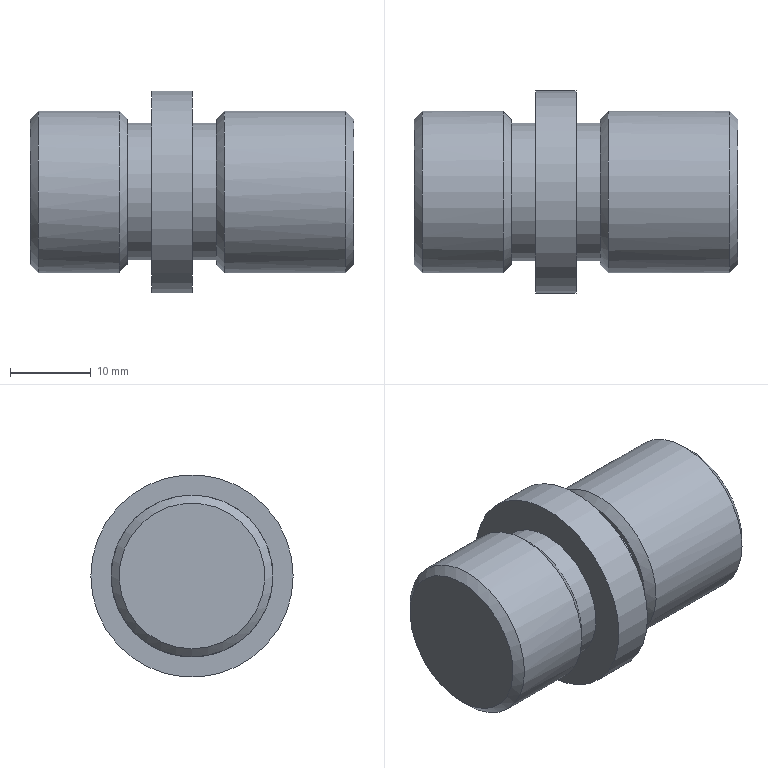Component | NX | MANDREL | 1 solid | 15 faces | box 40 x 25 x 25 mm | volume 12805 mm3 | plane 6 | cylinder 5 | cone 4 | commonest cylinder face diameters 17 x2 20 x2 25 x1
STEP:
#1=CARTESIAN_POINT('',(0.,0.,0.));
#2=DIRECTION('',(0.,0.,1.));
#3=DIRECTION('',(1.,0.,0.));
#4=AXIS2_PLACEMENT_3D('',#1,#2,#3);
#5=CARTESIAN_POINT('',(-22.,12.5,-57.));
#6=VERTEX_POINT('',#5);
#7=CARTESIAN_POINT('',(-22.,0.,-57.));
#8=DIRECTION('',(1.,0.,0.));
#9=DIRECTION('',(0.,1.,0.));
#10=AXIS2_PLACEMENT_3D('',#7,#8,#9);
#11=CIRCLE('',#10,12.5);
#12=CARTESIAN_POINT('',(-22.,0.,-57.));
#13=DIRECTION('',(-1.,0.,0.));
#14=DIRECTION('',(0.,0.,1.));
#15=AXIS2_PLACEMENT_3D('',#12,#13,#14);
#16=CYLINDRICAL_SURFACE('',#15,12.5);
#17=CARTESIAN_POINT('',(7.854,0.));
#18=DIRECTION('',(-1.,0.));
#19=VECTOR('',#18,1.);
#20=LINE('',#17,#19);
#21=(GEOMETRIC_REPRESENTATION_CONTEXT(2)PARAMETRIC_REPRESENTATION_CONTEXT()REPRESENTATION_CONTEXT('',''));
#22=DEFINITIONAL_REPRESENTATION('',(#20),#21);
#23=PCURVE('',#16,#22);
#24=CARTESIAN_POINT('',(-22.,0.,-57.));
#25=DIRECTION('',(1.,0.,0.));
#26=DIRECTION('',(0.,0.,-1.));
#27=AXIS2_PLACEMENT_3D('',#24,#25,#26);
#28=PLANE('',#27);
#29=CARTESIAN_POINT('',(0.,0.));
#30=DIRECTION('',(0.,1.));
#31=AXIS2_PLACEMENT_2D('',#29,#30);
#32=CIRCLE('',#31,12.5);
#33=(GEOMETRIC_REPRESENTATION_CONTEXT(2)PARAMETRIC_REPRESENTATION_CONTEXT()REPRESENTATION_CONTEXT('',''));
#34=DEFINITIONAL_REPRESENTATION('',(#32),#33);
#35=PCURVE('',#28,#34);
#36=SURFACE_CURVE('',#11,(#23,#35),.PCURVE_S1.);
#37=EDGE_CURVE('',#6,#6,#36,.T.);
#38=ORIENTED_EDGE('',*,*,#37,.F.);
#39=CARTESIAN_POINT('',(-27.,12.5,-57.));
#40=VERTEX_POINT('',#39);
#41=CARTESIAN_POINT('',(-22.,12.5,-57.));
#42=CARTESIAN_POINT('',(-27.,12.5,-57.));
#43=B_SPLINE_CURVE_WITH_KNOTS('',1,(#41,#42),.UNSPECIFIED.,.F.,.F.,(2,2),(0.,5.),.PIECEWISE_BEZIER_KNOTS.);
#44=CARTESIAN_POINT('',(7.854,0.));
#45=DIRECTION('',(0.,1.));
#46=VECTOR('',#45,1.);
#47=LINE('',#44,#46);
#48=(GEOMETRIC_REPRESENTATION_CONTEXT(2)PARAMETRIC_REPRESENTATION_CONTEXT()REPRESENTATION_CONTEXT('',''));
#49=DEFINITIONAL_REPRESENTATION('',(#47),#48);
#50=PCURVE('',#16,#49);
#51=CARTESIAN_POINT('',(1.571,0.));
#52=DIRECTION('',(0.,1.));
#53=VECTOR('',#52,1.);
#54=LINE('',#51,#53);
#55=(GEOMETRIC_REPRESENTATION_CONTEXT(2)PARAMETRIC_REPRESENTATION_CONTEXT()REPRESENTATION_CONTEXT('',''));
#56=DEFINITIONAL_REPRESENTATION('',(#54),#55);
#57=PCURVE('',#16,#56);
#58=SEAM_CURVE('',#43,(#50,#57),.PCURVE_S1.);
#59=EDGE_CURVE('',#6,#40,#58,.T.);
#60=ORIENTED_EDGE('',*,*,#59,.T.);
#61=CARTESIAN_POINT('',(-27.,0.,-57.));
#62=DIRECTION('',(1.,0.,0.));
#63=DIRECTION('',(0.,1.,0.));
#64=AXIS2_PLACEMENT_3D('',#61,#62,#63);
#65=CIRCLE('',#64,12.5);
#66=CARTESIAN_POINT('',(7.854,5.));
#67=DIRECTION('',(-1.,0.));
#68=VECTOR('',#67,1.);
#69=LINE('',#66,#68);
#70=(GEOMETRIC_REPRESENTATION_CONTEXT(2)PARAMETRIC_REPRESENTATION_CONTEXT()REPRESENTATION_CONTEXT('',''));
#71=DEFINITIONAL_REPRESENTATION('',(#69),#70);
#72=PCURVE('',#16,#71);
#73=CARTESIAN_POINT('',(-27.,0.,-57.));
#74=DIRECTION('',(1.,0.,0.));
#75=DIRECTION('',(0.,0.,-1.));
#76=AXIS2_PLACEMENT_3D('',#73,#74,#75);
#77=PLANE('',#76);
#78=CARTESIAN_POINT('',(0.,0.));
#79=DIRECTION('',(0.,1.));
#80=AXIS2_PLACEMENT_2D('',#78,#79);
#81=CIRCLE('',#80,12.5);
#82=(GEOMETRIC_REPRESENTATION_CONTEXT(2)PARAMETRIC_REPRESENTATION_CONTEXT()REPRESENTATION_CONTEXT('',''));
#83=DEFINITIONAL_REPRESENTATION('',(#81),#82);
#84=PCURVE('',#77,#83);
#85=SURFACE_CURVE('',#65,(#72,#84),.PCURVE_S1.);
#86=EDGE_CURVE('',#40,#40,#85,.T.);
#87=ORIENTED_EDGE('',*,*,#86,.T.);
#88=ORIENTED_EDGE('',*,*,#59,.F.);
#89=EDGE_LOOP('',(#38,#60,#87,#88));
#90=FACE_BOUND('',#89,.T.);
#91=ADVANCED_FACE('',(#90),#16,.T.);
#92=ORIENTED_EDGE('',*,*,#37,.T.);
#93=EDGE_LOOP('',(#92));
#94=FACE_BOUND('',#93,.T.);
#95=CARTESIAN_POINT('',(-22.,0.,-48.5));
#96=VERTEX_POINT('',#95);
#97=CARTESIAN_POINT('',(-22.,0.,-57.));
#98=DIRECTION('',(-1.,0.,0.));
#99=DIRECTION('',(0.,0.,1.));
#100=AXIS2_PLACEMENT_3D('',#97,#98,#99);
#101=CIRCLE('',#100,8.5);
#102=CARTESIAN_POINT('',(-8.5,0.));
#103=CARTESIAN_POINT('',(-8.5,14.722));
#104=CARTESIAN_POINT('',(4.25,7.361));
#105=CARTESIAN_POINT('',(17.,0.));
#106=CARTESIAN_POINT('',(4.25,-7.361));
#107=CARTESIAN_POINT('',(-8.5,-14.722));
#108=CARTESIAN_POINT('',(-8.5,0.));
#109=(BOUNDED_CURVE()B_SPLINE_CURVE(2,(#102,#103,#104,#105,#106,#107,#108),.UNSPECIFIED.,.T.,.F.)B_SPLINE_CURVE_WITH_KNOTS((1,2,2,2,2,1),(-2.094,0.,2.094,4.189,6.283,8.378),.UNSPECIFIED.)CURVE()GEOMETRIC_REPRESENTATION_ITEM()RATIONAL_B_SPLINE_CURVE((1.,0.5,1.,0.5,1.,0.5,1.))REPRESENTATION_ITEM(''));
#110=(GEOMETRIC_REPRESENTATION_CONTEXT(2)PARAMETRIC_REPRESENTATION_CONTEXT()REPRESENTATION_CONTEXT('',''));
#111=DEFINITIONAL_REPRESENTATION('',(#109),#110);
#112=PCURVE('',#28,#111);
#113=CARTESIAN_POINT('',(-20.5,0.,-57.));
#114=DIRECTION('',(-1.,0.,0.));
#115=DIRECTION('',(0.,0.,1.));
#116=AXIS2_PLACEMENT_3D('',#113,#114,#115);
#117=CYLINDRICAL_SURFACE('',#116,8.5);
#118=CARTESIAN_POINT('',(0.,1.5));
#119=DIRECTION('',(1.,0.));
#120=VECTOR('',#119,1.);
#121=LINE('',#118,#120);
#122=(GEOMETRIC_REPRESENTATION_CONTEXT(2)PARAMETRIC_REPRESENTATION_CONTEXT()REPRESENTATION_CONTEXT('',''));
#123=DEFINITIONAL_REPRESENTATION('',(#121),#122);
#124=PCURVE('',#117,#123);
#125=SURFACE_CURVE('',#101,(#112,#124),.PCURVE_S1.);
#126=EDGE_CURVE('',#96,#96,#125,.T.);
#127=ORIENTED_EDGE('',*,*,#126,.T.);
#128=EDGE_LOOP('',(#127));
#129=FACE_BOUND('',#128,.T.);
#130=ADVANCED_FACE('',(#94,#129),#28,.T.);
#131=ORIENTED_EDGE('',*,*,#86,.F.);
#132=EDGE_LOOP('',(#131));
#133=FACE_BOUND('',#132,.T.);
#134=CARTESIAN_POINT('',(-27.,0.,-48.5));
#135=VERTEX_POINT('',#134);
#136=CARTESIAN_POINT('',(-27.,0.,-57.));
#137=DIRECTION('',(-1.,0.,0.));
#138=DIRECTION('',(0.,0.,1.));
#139=AXIS2_PLACEMENT_3D('',#136,#137,#138);
#140=CIRCLE('',#139,8.5);
#141=CARTESIAN_POINT('',(-8.5,0.));
#142=CARTESIAN_POINT('',(-8.5,14.722));
#143=CARTESIAN_POINT('',(4.25,7.361));
#144=CARTESIAN_POINT('',(17.,0.));
#145=CARTESIAN_POINT('',(4.25,-7.361));
#146=CARTESIAN_POINT('',(-8.5,-14.722));
#147=CARTESIAN_POINT('',(-8.5,0.));
#148=(BOUNDED_CURVE()B_SPLINE_CURVE(2,(#141,#142,#143,#144,#145,#146,#147),.UNSPECIFIED.,.T.,.F.)B_SPLINE_CURVE_WITH_KNOTS((1,2,2,2,2,1),(-2.094,0.,2.094,4.189,6.283,8.378),.UNSPECIFIED.)CURVE()GEOMETRIC_REPRESENTATION_ITEM()RATIONAL_B_SPLINE_CURVE((1.,0.5,1.,0.5,1.,0.5,1.))REPRESENTATION_ITEM(''));
#149=(GEOMETRIC_REPRESENTATION_CONTEXT(2)PARAMETRIC_REPRESENTATION_CONTEXT()REPRESENTATION_CONTEXT('',''));
#150=DEFINITIONAL_REPRESENTATION('',(#148),#149);
#151=PCURVE('',#77,#150);
#152=CARTESIAN_POINT('',(-28.5,0.,-57.));
#153=DIRECTION('',(-1.,0.,0.));
#154=DIRECTION('',(0.,0.,1.));
#155=AXIS2_PLACEMENT_3D('',#152,#153,#154);
#156=CYLINDRICAL_SURFACE('',#155,8.5);
#157=CARTESIAN_POINT('',(0.,-1.5));
#158=DIRECTION('',(1.,0.));
#159=VECTOR('',#158,1.);
#160=LINE('',#157,#159);
#161=(GEOMETRIC_REPRESENTATION_CONTEXT(2)PARAMETRIC_REPRESENTATION_CONTEXT()REPRESENTATION_CONTEXT('',''));
#162=DEFINITIONAL_REPRESENTATION('',(#160),#161);
#163=PCURVE('',#156,#162);
#164=SURFACE_CURVE('',#140,(#151,#163),.PCURVE_S1.);
#165=EDGE_CURVE('',#135,#135,#164,.T.);
#166=ORIENTED_EDGE('',*,*,#165,.F.);
#167=EDGE_LOOP('',(#166));
#168=FACE_BOUND('',#167,.T.);
#169=ADVANCED_FACE('',(#133,#168),#77,.F.);
#170=CARTESIAN_POINT('',(-30.,0.,-48.));
#171=VERTEX_POINT('',#170);
#172=CARTESIAN_POINT('',(-30.,0.,-57.));
#173=DIRECTION('',(1.,0.,0.));
#174=DIRECTION('',(0.,0.,1.));
#175=AXIS2_PLACEMENT_3D('',#172,#173,#174);
#176=CIRCLE('',#175,9.);
#177=CARTESIAN_POINT('',(-30.,0.,-57.));
#178=DIRECTION('',(-1.,0.,0.));
#179=DIRECTION('',(0.,0.,1.));
#180=AXIS2_PLACEMENT_3D('',#177,#178,#179);
#181=PLANE('',#180);
#182=CARTESIAN_POINT('',(9.,0.));
#183=CARTESIAN_POINT('',(9.,-15.588));
#184=CARTESIAN_POINT('',(-4.5,-7.794));
#185=CARTESIAN_POINT('',(-18.,-0.));
#186=CARTESIAN_POINT('',(-4.5,7.794));
#187=CARTESIAN_POINT('',(9.,15.588));
#188=CARTESIAN_POINT('',(9.,0.));
#189=(BOUNDED_CURVE()B_SPLINE_CURVE(2,(#182,#183,#184,#185,#186,#187,#188),.UNSPECIFIED.,.T.,.F.)B_SPLINE_CURVE_WITH_KNOTS((1,2,2,2,2,1),(-2.094,0.,2.094,4.189,6.283,8.378),.UNSPECIFIED.)CURVE()GEOMETRIC_REPRESENTATION_ITEM()RATIONAL_B_SPLINE_CURVE((1.,0.5,1.,0.5,1.,0.5,1.))REPRESENTATION_ITEM(''));
#190=(GEOMETRIC_REPRESENTATION_CONTEXT(2)PARAMETRIC_REPRESENTATION_CONTEXT()REPRESENTATION_CONTEXT('',''));
#191=DEFINITIONAL_REPRESENTATION('',(#189),#190);
#192=PCURVE('',#181,#191);
#193=CARTESIAN_POINT('',(-31.,0.,-57.));
#194=DIRECTION('',(-1.,0.,0.));
#195=DIRECTION('',(0.,0.,1.));
#196=AXIS2_PLACEMENT_3D('',#193,#194,#195);
#197=CONICAL_SURFACE('',#196,10.,0.7854);
#198=CARTESIAN_POINT('',(6.283,-1.));
#199=DIRECTION('',(-1.,0.));
#200=VECTOR('',#199,1.);
#201=LINE('',#198,#200);
#202=(GEOMETRIC_REPRESENTATION_CONTEXT(2)PARAMETRIC_REPRESENTATION_CONTEXT()REPRESENTATION_CONTEXT('',''));
#203=DEFINITIONAL_REPRESENTATION('',(#201),#202);
#204=PCURVE('',#197,#203);
#205=SURFACE_CURVE('',#176,(#192,#204),.PCURVE_S1.);
#206=EDGE_CURVE('',#171,#171,#205,.T.);
#207=ORIENTED_EDGE('',*,*,#206,.T.);
#208=EDGE_LOOP('',(#207));
#209=FACE_BOUND('',#208,.T.);
#210=CARTESIAN_POINT('',(-30.,0.,-48.5));
#211=VERTEX_POINT('',#210);
#212=CARTESIAN_POINT('',(-30.,0.,-57.));
#213=DIRECTION('',(1.,0.,0.));
#214=DIRECTION('',(0.,0.,1.));
#215=AXIS2_PLACEMENT_3D('',#212,#213,#214);
#216=CIRCLE('',#215,8.5);
#217=CARTESIAN_POINT('',(8.5,0.));
#218=CARTESIAN_POINT('',(8.5,-14.722));
#219=CARTESIAN_POINT('',(-4.25,-7.361));
#220=CARTESIAN_POINT('',(-17.,-0.));
#221=CARTESIAN_POINT('',(-4.25,7.361));
#222=CARTESIAN_POINT('',(8.5,14.722));
#223=CARTESIAN_POINT('',(8.5,0.));
#224=(BOUNDED_CURVE()B_SPLINE_CURVE(2,(#217,#218,#219,#220,#221,#222,#223),.UNSPECIFIED.,.T.,.F.)B_SPLINE_CURVE_WITH_KNOTS((1,2,2,2,2,1),(-2.094,0.,2.094,4.189,6.283,8.378),.UNSPECIFIED.)CURVE()GEOMETRIC_REPRESENTATION_ITEM()RATIONAL_B_SPLINE_CURVE((1.,0.5,1.,0.5,1.,0.5,1.))REPRESENTATION_ITEM(''));
#225=(GEOMETRIC_REPRESENTATION_CONTEXT(2)PARAMETRIC_REPRESENTATION_CONTEXT()REPRESENTATION_CONTEXT('',''));
#226=DEFINITIONAL_REPRESENTATION('',(#224),#225);
#227=PCURVE('',#181,#226);
#228=CARTESIAN_POINT('',(6.283,1.5));
#229=DIRECTION('',(-1.,0.));
#230=VECTOR('',#229,1.);
#231=LINE('',#228,#230);
#232=(GEOMETRIC_REPRESENTATION_CONTEXT(2)PARAMETRIC_REPRESENTATION_CONTEXT()REPRESENTATION_CONTEXT('',''));
#233=DEFINITIONAL_REPRESENTATION('',(#231),#232);
#234=PCURVE('',#156,#233);
#235=SURFACE_CURVE('',#216,(#227,#234),.PCURVE_S1.);
#236=EDGE_CURVE('',#211,#211,#235,.T.);
#237=ORIENTED_EDGE('',*,*,#236,.F.);
#238=EDGE_LOOP('',(#237));
#239=FACE_BOUND('',#238,.T.);
#240=ADVANCED_FACE('',(#209,#239),#181,.F.);
#241=ORIENTED_EDGE('',*,*,#236,.T.);
#242=CARTESIAN_POINT('',(-27.,-0.,-48.5));
#243=CARTESIAN_POINT('',(-30.,-0.,-48.5));
#244=B_SPLINE_CURVE_WITH_KNOTS('',1,(#242,#243),.UNSPECIFIED.,.F.,.F.,(2,2),(-1.5,1.5),.PIECEWISE_BEZIER_KNOTS.);
#245=CARTESIAN_POINT('',(0.,0.));
#246=DIRECTION('',(0.,1.));
#247=VECTOR('',#246,1.);
#248=LINE('',#245,#247);
#249=(GEOMETRIC_REPRESENTATION_CONTEXT(2)PARAMETRIC_REPRESENTATION_CONTEXT()REPRESENTATION_CONTEXT('',''));
#250=DEFINITIONAL_REPRESENTATION('',(#248),#249);
#251=PCURVE('',#156,#250);
#252=CARTESIAN_POINT('',(6.283,0.));
#253=DIRECTION('',(0.,1.));
#254=VECTOR('',#253,1.);
#255=LINE('',#252,#254);
#256=(GEOMETRIC_REPRESENTATION_CONTEXT(2)PARAMETRIC_REPRESENTATION_CONTEXT()REPRESENTATION_CONTEXT('',''));
#257=DEFINITIONAL_REPRESENTATION('',(#255),#256);
#258=PCURVE('',#156,#257);
#259=SEAM_CURVE('',#244,(#251,#258),.PCURVE_S1.);
#260=EDGE_CURVE('',#135,#211,#259,.T.);
#261=ORIENTED_EDGE('',*,*,#260,.F.);
#262=ORIENTED_EDGE('',*,*,#165,.T.);
#263=ORIENTED_EDGE('',*,*,#260,.T.);
#264=EDGE_LOOP('',(#241,#261,#262,#263));
#265=FACE_BOUND('',#264,.T.);
#266=ADVANCED_FACE('',(#265),#156,.T.);
#267=CARTESIAN_POINT('',(-42.,0.,-66.));
#268=VERTEX_POINT('',#267);
#269=CARTESIAN_POINT('',(-42.,0.,-57.));
#270=DIRECTION('',(-1.,0.,0.));
#271=DIRECTION('',(0.,0.,-1.));
#272=AXIS2_PLACEMENT_3D('',#269,#270,#271);
#273=CIRCLE('',#272,9.);
#274=CARTESIAN_POINT('',(-42.,0.,-57.));
#275=DIRECTION('',(1.,0.,0.));
#276=DIRECTION('',(0.,0.,-1.));
#277=AXIS2_PLACEMENT_3D('',#274,#275,#276);
#278=PLANE('',#277);
#279=CARTESIAN_POINT('',(9.,0.));
#280=CARTESIAN_POINT('',(9.,-15.588));
#281=CARTESIAN_POINT('',(-4.5,-7.794));
#282=CARTESIAN_POINT('',(-18.,-0.));
#283=CARTESIAN_POINT('',(-4.5,7.794));
#284=CARTESIAN_POINT('',(9.,15.588));
#285=CARTESIAN_POINT('',(9.,0.));
#286=(BOUNDED_CURVE()B_SPLINE_CURVE(2,(#279,#280,#281,#282,#283,#284,#285),.UNSPECIFIED.,.T.,.F.)B_SPLINE_CURVE_WITH_KNOTS((1,2,2,2,2,1),(-2.094,0.,2.094,4.189,6.283,8.378),.UNSPECIFIED.)CURVE()GEOMETRIC_REPRESENTATION_ITEM()RATIONAL_B_SPLINE_CURVE((1.,0.5,1.,0.5,1.,0.5,1.))REPRESENTATION_ITEM(''));
#287=(GEOMETRIC_REPRESENTATION_CONTEXT(2)PARAMETRIC_REPRESENTATION_CONTEXT()REPRESENTATION_CONTEXT('',''));
#288=DEFINITIONAL_REPRESENTATION('',(#286),#287);
#289=PCURVE('',#278,#288);
#290=CARTESIAN_POINT('',(-41.,0.,-57.));
#291=DIRECTION('',(1.,0.,0.));
#292=DIRECTION('',(0.,0.,-1.));
#293=AXIS2_PLACEMENT_3D('',#290,#291,#292);
#294=CONICAL_SURFACE('',#293,10.,0.7854);
#295=CARTESIAN_POINT('',(6.283,-1.));
#296=DIRECTION('',(-1.,0.));
#297=VECTOR('',#296,1.);
#298=LINE('',#295,#297);
#299=(GEOMETRIC_REPRESENTATION_CONTEXT(2)PARAMETRIC_REPRESENTATION_CONTEXT()REPRESENTATION_CONTEXT('',''));
#300=DEFINITIONAL_REPRESENTATION('',(#298),#299);
#301=PCURVE('',#294,#300);
#302=SURFACE_CURVE('',#273,(#289,#301),.PCURVE_S1.);
#303=EDGE_CURVE('',#268,#268,#302,.T.);
#304=ORIENTED_EDGE('',*,*,#303,.T.);
#305=EDGE_LOOP('',(#304));
#306=FACE_BOUND('',#305,.T.);
#307=ADVANCED_FACE('',(#306),#278,.F.);
#308=CARTESIAN_POINT('',(-31.,0.,-47.));
#309=VERTEX_POINT('',#308);
#310=CARTESIAN_POINT('',(-31.,0.,-57.));
#311=DIRECTION('',(-1.,0.,0.));
#312=DIRECTION('',(0.,0.,1.));
#313=AXIS2_PLACEMENT_3D('',#310,#311,#312);
#314=CIRCLE('',#313,10.);
#315=CARTESIAN_POINT('',(-27.,0.,-57.));
#316=DIRECTION('',(-1.,0.,0.));
#317=DIRECTION('',(0.,0.,1.));
#318=AXIS2_PLACEMENT_3D('',#315,#316,#317);
#319=CYLINDRICAL_SURFACE('',#318,10.);
#320=CARTESIAN_POINT('',(0.,4.));
#321=DIRECTION('',(1.,0.));
#322=VECTOR('',#321,1.);
#323=LINE('',#320,#322);
#324=(GEOMETRIC_REPRESENTATION_CONTEXT(2)PARAMETRIC_REPRESENTATION_CONTEXT()REPRESENTATION_CONTEXT('',''));
#325=DEFINITIONAL_REPRESENTATION('',(#323),#324);
#326=PCURVE('',#319,#325);
#327=CARTESIAN_POINT('',(0.,0.));
#328=DIRECTION('',(1.,0.));
#329=VECTOR('',#328,1.);
#330=LINE('',#327,#329);
#331=(GEOMETRIC_REPRESENTATION_CONTEXT(2)PARAMETRIC_REPRESENTATION_CONTEXT()REPRESENTATION_CONTEXT('',''));
#332=DEFINITIONAL_REPRESENTATION('',(#330),#331);
#333=PCURVE('',#197,#332);
#334=SURFACE_CURVE('',#314,(#326,#333),.PCURVE_S1.);
#335=EDGE_CURVE('',#309,#309,#334,.T.);
#336=ORIENTED_EDGE('',*,*,#335,.T.);
#337=CARTESIAN_POINT('',(-41.,0.,-47.));
#338=VERTEX_POINT('',#337);
#339=CARTESIAN_POINT('',(-31.,0.,-47.));
#340=CARTESIAN_POINT('',(-41.,0.,-47.));
#341=B_SPLINE_CURVE_WITH_KNOTS('',1,(#339,#340),.UNSPECIFIED.,.F.,.F.,(2,2),(4.,14.),.PIECEWISE_BEZIER_KNOTS.);
#342=CARTESIAN_POINT('',(6.283,0.));
#343=DIRECTION('',(0.,1.));
#344=VECTOR('',#343,1.);
#345=LINE('',#342,#344);
#346=(GEOMETRIC_REPRESENTATION_CONTEXT(2)PARAMETRIC_REPRESENTATION_CONTEXT()REPRESENTATION_CONTEXT('',''));
#347=DEFINITIONAL_REPRESENTATION('',(#345),#346);
#348=PCURVE('',#319,#347);
#349=CARTESIAN_POINT('',(0.,0.));
#350=DIRECTION('',(0.,1.));
#351=VECTOR('',#350,1.);
#352=LINE('',#349,#351);
#353=(GEOMETRIC_REPRESENTATION_CONTEXT(2)PARAMETRIC_REPRESENTATION_CONTEXT()REPRESENTATION_CONTEXT('',''));
#354=DEFINITIONAL_REPRESENTATION('',(#352),#353);
#355=PCURVE('',#319,#354);
#356=SEAM_CURVE('',#341,(#348,#355),.PCURVE_S1.);
#357=EDGE_CURVE('',#309,#338,#356,.T.);
#358=ORIENTED_EDGE('',*,*,#357,.T.);
#359=CARTESIAN_POINT('',(-41.,0.,-67.));
#360=VERTEX_POINT('',#359);
#361=CARTESIAN_POINT('',(-41.,0.,-57.));
#362=DIRECTION('',(1.,0.,0.));
#363=DIRECTION('',(0.,0.,-1.));
#364=AXIS2_PLACEMENT_3D('',#361,#362,#363);
#365=CIRCLE('',#364,10.);
#366=CARTESIAN_POINT('',(9.425,14.));
#367=DIRECTION('',(-1.,0.));
#368=VECTOR('',#367,1.);
#369=LINE('',#366,#368);
#370=(GEOMETRIC_REPRESENTATION_CONTEXT(2)PARAMETRIC_REPRESENTATION_CONTEXT()REPRESENTATION_CONTEXT('',''));
#371=DEFINITIONAL_REPRESENTATION('',(#369),#370);
#372=PCURVE('',#319,#371);
#373=CARTESIAN_POINT('',(0.,0.));
#374=DIRECTION('',(1.,0.));
#375=VECTOR('',#374,1.);
#376=LINE('',#373,#375);
#377=(GEOMETRIC_REPRESENTATION_CONTEXT(2)PARAMETRIC_REPRESENTATION_CONTEXT()REPRESENTATION_CONTEXT('',''));
#378=DEFINITIONAL_REPRESENTATION('',(#376),#377);
#379=PCURVE('',#294,#378);
#380=SURFACE_CURVE('',#365,(#372,#379),.PCURVE_S1.);
#381=EDGE_CURVE('',#338,#360,#380,.T.);
#382=ORIENTED_EDGE('',*,*,#381,.T.);
#383=CARTESIAN_POINT('',(-41.,0.,-57.));
#384=DIRECTION('',(1.,0.,0.));
#385=DIRECTION('',(0.,0.,-1.));
#386=AXIS2_PLACEMENT_3D('',#383,#384,#385);
#387=CIRCLE('',#386,10.);
#388=CARTESIAN_POINT('',(3.142,14.));
#389=DIRECTION('',(-1.,0.));
#390=VECTOR('',#389,1.);
#391=LINE('',#388,#390);
#392=(GEOMETRIC_REPRESENTATION_CONTEXT(2)PARAMETRIC_REPRESENTATION_CONTEXT()REPRESENTATION_CONTEXT('',''));
#393=DEFINITIONAL_REPRESENTATION('',(#391),#392);
#394=PCURVE('',#319,#393);
#395=CARTESIAN_POINT('',(0.,0.));
#396=DIRECTION('',(1.,0.));
#397=VECTOR('',#396,1.);
#398=LINE('',#395,#397);
#399=(GEOMETRIC_REPRESENTATION_CONTEXT(2)PARAMETRIC_REPRESENTATION_CONTEXT()REPRESENTATION_CONTEXT('',''));
#400=DEFINITIONAL_REPRESENTATION('',(#398),#399);
#401=PCURVE('',#294,#400);
#402=SURFACE_CURVE('',#387,(#394,#401),.PCURVE_S1.);
#403=EDGE_CURVE('',#360,#338,#402,.T.);
#404=ORIENTED_EDGE('',*,*,#403,.T.);
#405=ORIENTED_EDGE('',*,*,#357,.F.);
#406=EDGE_LOOP('',(#336,#358,#382,#404,#405));
#407=FACE_BOUND('',#406,.T.);
#408=ADVANCED_FACE('',(#407),#319,.T.);
#409=CARTESIAN_POINT('',(-19.,0.,-48.));
#410=VERTEX_POINT('',#409);
#411=CARTESIAN_POINT('',(-19.,0.,-57.));
#412=DIRECTION('',(-1.,0.,0.));
#413=DIRECTION('',(0.,0.,1.));
#414=AXIS2_PLACEMENT_3D('',#411,#412,#413);
#415=CIRCLE('',#414,9.);
#416=CARTESIAN_POINT('',(-19.,0.,-57.));
#417=DIRECTION('',(-1.,0.,0.));
#418=DIRECTION('',(0.,0.,1.));
#419=AXIS2_PLACEMENT_3D('',#416,#417,#418);
#420=PLANE('',#419);
#421=CARTESIAN_POINT('',(0.,0.));
#422=DIRECTION('',(1.,0.));
#423=AXIS2_PLACEMENT_2D('',#421,#422);
#424=CIRCLE('',#423,9.);
#425=(GEOMETRIC_REPRESENTATION_CONTEXT(2)PARAMETRIC_REPRESENTATION_CONTEXT()REPRESENTATION_CONTEXT('',''));
#426=DEFINITIONAL_REPRESENTATION('',(#424),#425);
#427=PCURVE('',#420,#426);
#428=CARTESIAN_POINT('',(-19.,0.,-57.));
#429=DIRECTION('',(1.,0.,0.));
#430=DIRECTION('',(0.,0.,-1.));
#431=AXIS2_PLACEMENT_3D('',#428,#429,#430);
#432=CONICAL_SURFACE('',#431,9.,0.7854);
#433=CARTESIAN_POINT('',(9.425,0.));
#434=DIRECTION('',(-1.,0.));
#435=VECTOR('',#434,1.);
#436=LINE('',#433,#435);
#437=(GEOMETRIC_REPRESENTATION_CONTEXT(2)PARAMETRIC_REPRESENTATION_CONTEXT()REPRESENTATION_CONTEXT('',''));
#438=DEFINITIONAL_REPRESENTATION('',(#436),#437);
#439=PCURVE('',#432,#438);
#440=SURFACE_CURVE('',#415,(#427,#439),.PCURVE_S1.);
#441=EDGE_CURVE('',#410,#410,#440,.T.);
#442=ORIENTED_EDGE('',*,*,#441,.T.);
#443=EDGE_LOOP('',(#442));
#444=FACE_BOUND('',#443,.T.);
#445=CARTESIAN_POINT('',(-19.,0.,-48.5));
#446=VERTEX_POINT('',#445);
#447=CARTESIAN_POINT('',(-19.,0.,-57.));
#448=DIRECTION('',(1.,0.,0.));
#449=DIRECTION('',(0.,0.,1.));
#450=AXIS2_PLACEMENT_3D('',#447,#448,#449);
#451=CIRCLE('',#450,8.5);
#452=CARTESIAN_POINT('',(8.5,0.));
#453=CARTESIAN_POINT('',(8.5,-14.722));
#454=CARTESIAN_POINT('',(-4.25,-7.361));
#455=CARTESIAN_POINT('',(-17.,-0.));
#456=CARTESIAN_POINT('',(-4.25,7.361));
#457=CARTESIAN_POINT('',(8.5,14.722));
#458=CARTESIAN_POINT('',(8.5,0.));
#459=(BOUNDED_CURVE()B_SPLINE_CURVE(2,(#452,#453,#454,#455,#456,#457,#458),.UNSPECIFIED.,.T.,.F.)B_SPLINE_CURVE_WITH_KNOTS((1,2,2,2,2,1),(-2.094,0.,2.094,4.189,6.283,8.378),.UNSPECIFIED.)CURVE()GEOMETRIC_REPRESENTATION_ITEM()RATIONAL_B_SPLINE_CURVE((1.,0.5,1.,0.5,1.,0.5,1.))REPRESENTATION_ITEM(''));
#460=(GEOMETRIC_REPRESENTATION_CONTEXT(2)PARAMETRIC_REPRESENTATION_CONTEXT()REPRESENTATION_CONTEXT('',''));
#461=DEFINITIONAL_REPRESENTATION('',(#459),#460);
#462=PCURVE('',#420,#461);
#463=CARTESIAN_POINT('',(6.283,-1.5));
#464=DIRECTION('',(-1.,0.));
#465=VECTOR('',#464,1.);
#466=LINE('',#463,#465);
#467=(GEOMETRIC_REPRESENTATION_CONTEXT(2)PARAMETRIC_REPRESENTATION_CONTEXT()REPRESENTATION_CONTEXT('',''));
#468=DEFINITIONAL_REPRESENTATION('',(#466),#467);
#469=PCURVE('',#117,#468);
#470=SURFACE_CURVE('',#451,(#462,#469),.PCURVE_S1.);
#471=EDGE_CURVE('',#446,#446,#470,.T.);
#472=ORIENTED_EDGE('',*,*,#471,.T.);
#473=EDGE_LOOP('',(#472));
#474=FACE_BOUND('',#473,.T.);
#475=ADVANCED_FACE('',(#444,#474),#420,.T.);
#476=ORIENTED_EDGE('',*,*,#126,.F.);
#477=CARTESIAN_POINT('',(-19.,-0.,-48.5));
#478=CARTESIAN_POINT('',(-22.,-0.,-48.5));
#479=B_SPLINE_CURVE_WITH_KNOTS('',1,(#477,#478),.UNSPECIFIED.,.F.,.F.,(2,2),(-1.5,1.5),.PIECEWISE_BEZIER_KNOTS.);
#480=CARTESIAN_POINT('',(0.,0.));
#481=DIRECTION('',(0.,1.));
#482=VECTOR('',#481,1.);
#483=LINE('',#480,#482);
#484=(GEOMETRIC_REPRESENTATION_CONTEXT(2)PARAMETRIC_REPRESENTATION_CONTEXT()REPRESENTATION_CONTEXT('',''));
#485=DEFINITIONAL_REPRESENTATION('',(#483),#484);
#486=PCURVE('',#117,#485);
#487=CARTESIAN_POINT('',(6.283,0.));
#488=DIRECTION('',(0.,1.));
#489=VECTOR('',#488,1.);
#490=LINE('',#487,#489);
#491=(GEOMETRIC_REPRESENTATION_CONTEXT(2)PARAMETRIC_REPRESENTATION_CONTEXT()REPRESENTATION_CONTEXT('',''));
#492=DEFINITIONAL_REPRESENTATION('',(#490),#491);
#493=PCURVE('',#117,#492);
#494=SEAM_CURVE('',#479,(#486,#493),.PCURVE_S1.);
#495=EDGE_CURVE('',#446,#96,#494,.T.);
#496=ORIENTED_EDGE('',*,*,#495,.F.);
#497=ORIENTED_EDGE('',*,*,#471,.F.);
#498=ORIENTED_EDGE('',*,*,#495,.T.);
#499=EDGE_LOOP('',(#476,#496,#497,#498));
#500=FACE_BOUND('',#499,.T.);
#501=ADVANCED_FACE('',(#500),#117,.T.);
#502=CARTESIAN_POINT('',(-2.,0.,-66.));
#503=VERTEX_POINT('',#502);
#504=CARTESIAN_POINT('',(-2.,0.,-57.));
#505=DIRECTION('',(1.,0.,0.));
#506=DIRECTION('',(0.,0.,-1.));
#507=AXIS2_PLACEMENT_3D('',#504,#505,#506);
#508=CIRCLE('',#507,9.);
#509=CARTESIAN_POINT('',(-2.,0.,-57.));
#510=DIRECTION('',(1.,0.,0.));
#511=DIRECTION('',(0.,0.,-1.));
#512=AXIS2_PLACEMENT_3D('',#509,#510,#511);
#513=PLANE('',#512);
#514=CARTESIAN_POINT('',(0.,0.));
#515=DIRECTION('',(1.,0.));
#516=AXIS2_PLACEMENT_2D('',#514,#515);
#517=CIRCLE('',#516,9.);
#518=(GEOMETRIC_REPRESENTATION_CONTEXT(2)PARAMETRIC_REPRESENTATION_CONTEXT()REPRESENTATION_CONTEXT('',''));
#519=DEFINITIONAL_REPRESENTATION('',(#517),#518);
#520=PCURVE('',#513,#519);
#521=CARTESIAN_POINT('',(-2.,0.,-57.));
#522=DIRECTION('',(-1.,0.,0.));
#523=DIRECTION('',(0.,0.,1.));
#524=AXIS2_PLACEMENT_3D('',#521,#522,#523);
#525=CONICAL_SURFACE('',#524,9.,0.7854);
#526=CARTESIAN_POINT('',(9.425,0.));
#527=DIRECTION('',(-1.,0.));
#528=VECTOR('',#527,1.);
#529=LINE('',#526,#528);
#530=(GEOMETRIC_REPRESENTATION_CONTEXT(2)PARAMETRIC_REPRESENTATION_CONTEXT()REPRESENTATION_CONTEXT('',''));
#531=DEFINITIONAL_REPRESENTATION('',(#529),#530);
#532=PCURVE('',#525,#531);
#533=SURFACE_CURVE('',#508,(#520,#532),.PCURVE_S1.);
#534=EDGE_CURVE('',#503,#503,#533,.T.);
#535=ORIENTED_EDGE('',*,*,#534,.T.);
#536=EDGE_LOOP('',(#535));
#537=FACE_BOUND('',#536,.T.);
#538=ADVANCED_FACE('',(#537),#513,.T.);
#539=CARTESIAN_POINT('',(-18.,0.,-47.));
#540=VERTEX_POINT('',#539);
#541=CARTESIAN_POINT('',(-18.,0.,-57.));
#542=DIRECTION('',(1.,0.,0.));
#543=DIRECTION('',(0.,0.,1.));
#544=AXIS2_PLACEMENT_3D('',#541,#542,#543);
#545=CIRCLE('',#544,10.);
#546=CARTESIAN_POINT('',(-2.,0.,-57.));
#547=DIRECTION('',(-1.,0.,0.));
#548=DIRECTION('',(0.,0.,1.));
#549=AXIS2_PLACEMENT_3D('',#546,#547,#548);
#550=CYLINDRICAL_SURFACE('',#549,10.);
#551=CARTESIAN_POINT('',(6.283,16.));
#552=DIRECTION('',(-1.,0.));
#553=VECTOR('',#552,1.);
#554=LINE('',#551,#553);
#555=(GEOMETRIC_REPRESENTATION_CONTEXT(2)PARAMETRIC_REPRESENTATION_CONTEXT()REPRESENTATION_CONTEXT('',''));
#556=DEFINITIONAL_REPRESENTATION('',(#554),#555);
#557=PCURVE('',#550,#556);
#558=CARTESIAN_POINT('',(3.142,1.));
#559=DIRECTION('',(1.,0.));
#560=VECTOR('',#559,1.);
#561=LINE('',#558,#560);
#562=(GEOMETRIC_REPRESENTATION_CONTEXT(2)PARAMETRIC_REPRESENTATION_CONTEXT()REPRESENTATION_CONTEXT('',''));
#563=DEFINITIONAL_REPRESENTATION('',(#561),#562);
#564=PCURVE('',#432,#563);
#565=SURFACE_CURVE('',#545,(#557,#564),.PCURVE_S1.);
#566=EDGE_CURVE('',#540,#540,#565,.T.);
#567=ORIENTED_EDGE('',*,*,#566,.T.);
#568=CARTESIAN_POINT('',(-3.,-0.,-47.));
#569=VERTEX_POINT('',#568);
#570=CARTESIAN_POINT('',(-3.,-0.,-47.));
#571=CARTESIAN_POINT('',(-18.,-0.,-47.));
#572=B_SPLINE_CURVE_WITH_KNOTS('',1,(#570,#571),.UNSPECIFIED.,.F.,.F.,(2,2),(1.,16.),.PIECEWISE_BEZIER_KNOTS.);
#573=CARTESIAN_POINT('',(0.,0.));
#574=DIRECTION('',(0.,1.));
#575=VECTOR('',#574,1.);
#576=LINE('',#573,#575);
#577=(GEOMETRIC_REPRESENTATION_CONTEXT(2)PARAMETRIC_REPRESENTATION_CONTEXT()REPRESENTATION_CONTEXT('',''));
#578=DEFINITIONAL_REPRESENTATION('',(#576),#577);
#579=PCURVE('',#550,#578);
#580=CARTESIAN_POINT('',(6.283,0.));
#581=DIRECTION('',(0.,1.));
#582=VECTOR('',#581,1.);
#583=LINE('',#580,#582);
#584=(GEOMETRIC_REPRESENTATION_CONTEXT(2)PARAMETRIC_REPRESENTATION_CONTEXT()REPRESENTATION_CONTEXT('',''));
#585=DEFINITIONAL_REPRESENTATION('',(#583),#584);
#586=PCURVE('',#550,#585);
#587=SEAM_CURVE('',#572,(#579,#586),.PCURVE_S1.);
#588=EDGE_CURVE('',#569,#540,#587,.T.);
#589=ORIENTED_EDGE('',*,*,#588,.F.);
#590=CARTESIAN_POINT('',(-3.,0.,-67.));
#591=VERTEX_POINT('',#590);
#592=CARTESIAN_POINT('',(-3.,0.,-57.));
#593=DIRECTION('',(-1.,0.,0.));
#594=DIRECTION('',(0.,0.,-1.));
#595=AXIS2_PLACEMENT_3D('',#592,#593,#594);
#596=CIRCLE('',#595,10.);
#597=CARTESIAN_POINT('',(-3.142,1.));
#598=DIRECTION('',(1.,0.));
#599=VECTOR('',#598,1.);
#600=LINE('',#597,#599);
#601=(GEOMETRIC_REPRESENTATION_CONTEXT(2)PARAMETRIC_REPRESENTATION_CONTEXT()REPRESENTATION_CONTEXT('',''));
#602=DEFINITIONAL_REPRESENTATION('',(#600),#601);
#603=PCURVE('',#550,#602);
#604=CARTESIAN_POINT('',(3.142,1.));
#605=DIRECTION('',(1.,0.));
#606=VECTOR('',#605,1.);
#607=LINE('',#604,#606);
#608=(GEOMETRIC_REPRESENTATION_CONTEXT(2)PARAMETRIC_REPRESENTATION_CONTEXT()REPRESENTATION_CONTEXT('',''));
#609=DEFINITIONAL_REPRESENTATION('',(#607),#608);
#610=PCURVE('',#525,#609);
#611=SURFACE_CURVE('',#596,(#603,#610),.PCURVE_S1.);
#612=EDGE_CURVE('',#569,#591,#611,.T.);
#613=ORIENTED_EDGE('',*,*,#612,.T.);
#614=CARTESIAN_POINT('',(-3.,0.,-57.));
#615=DIRECTION('',(-1.,0.,0.));
#616=DIRECTION('',(0.,0.,-1.));
#617=AXIS2_PLACEMENT_3D('',#614,#615,#616);
#618=CIRCLE('',#617,10.);
#619=CARTESIAN_POINT('',(3.142,1.));
#620=DIRECTION('',(1.,0.));
#621=VECTOR('',#620,1.);
#622=LINE('',#619,#621);
#623=(GEOMETRIC_REPRESENTATION_CONTEXT(2)PARAMETRIC_REPRESENTATION_CONTEXT()REPRESENTATION_CONTEXT('',''));
#624=DEFINITIONAL_REPRESENTATION('',(#622),#623);
#625=PCURVE('',#550,#624);
#626=CARTESIAN_POINT('',(3.142,1.));
#627=DIRECTION('',(1.,0.));
#628=VECTOR('',#627,1.);
#629=LINE('',#626,#628);
#630=(GEOMETRIC_REPRESENTATION_CONTEXT(2)PARAMETRIC_REPRESENTATION_CONTEXT()REPRESENTATION_CONTEXT('',''));
#631=DEFINITIONAL_REPRESENTATION('',(#629),#630);
#632=PCURVE('',#525,#631);
#633=SURFACE_CURVE('',#618,(#625,#632),.PCURVE_S1.);
#634=EDGE_CURVE('',#591,#569,#633,.T.);
#635=ORIENTED_EDGE('',*,*,#634,.T.);
#636=ORIENTED_EDGE('',*,*,#588,.T.);
#637=EDGE_LOOP('',(#567,#589,#613,#635,#636));
#638=FACE_BOUND('',#637,.T.);
#639=ADVANCED_FACE('',(#638),#550,.T.);
#640=ORIENTED_EDGE('',*,*,#566,.F.);
#641=CARTESIAN_POINT('',(-19.,0.,-48.));
#642=CARTESIAN_POINT('',(-18.,0.,-47.));
#643=B_SPLINE_CURVE_WITH_KNOTS('',1,(#641,#642),.UNSPECIFIED.,.F.,.F.,(2,2),(0.,1.414),.PIECEWISE_BEZIER_KNOTS.);
#644=CARTESIAN_POINT('',(3.142,0.));
#645=DIRECTION('',(0.,1.));
#646=VECTOR('',#645,1.);
#647=LINE('',#644,#646);
#648=(GEOMETRIC_REPRESENTATION_CONTEXT(2)PARAMETRIC_REPRESENTATION_CONTEXT()REPRESENTATION_CONTEXT('',''));
#649=DEFINITIONAL_REPRESENTATION('',(#647),#648);
#650=PCURVE('',#432,#649);
#651=CARTESIAN_POINT('',(9.425,0.));
#652=DIRECTION('',(0.,1.));
#653=VECTOR('',#652,1.);
#654=LINE('',#651,#653);
#655=(GEOMETRIC_REPRESENTATION_CONTEXT(2)PARAMETRIC_REPRESENTATION_CONTEXT()REPRESENTATION_CONTEXT('',''));
#656=DEFINITIONAL_REPRESENTATION('',(#654),#655);
#657=PCURVE('',#432,#656);
#658=SEAM_CURVE('',#643,(#650,#657),.PCURVE_S1.);
#659=EDGE_CURVE('',#410,#540,#658,.T.);
#660=ORIENTED_EDGE('',*,*,#659,.F.);
#661=ORIENTED_EDGE('',*,*,#441,.F.);
#662=ORIENTED_EDGE('',*,*,#659,.T.);
#663=EDGE_LOOP('',(#640,#660,#661,#662));
#664=FACE_BOUND('',#663,.T.);
#665=ADVANCED_FACE('',(#664),#432,.T.);
#666=ORIENTED_EDGE('',*,*,#206,.F.);
#667=CARTESIAN_POINT('',(-30.,0.,-48.));
#668=CARTESIAN_POINT('',(-31.,0.,-47.));
#669=B_SPLINE_CURVE_WITH_KNOTS('',1,(#667,#668),.UNSPECIFIED.,.F.,.F.,(2,2),(-1.414,0.),.PIECEWISE_BEZIER_KNOTS.);
#670=CARTESIAN_POINT('',(6.283,0.));
#671=DIRECTION('',(0.,1.));
#672=VECTOR('',#671,1.);
#673=LINE('',#670,#672);
#674=(GEOMETRIC_REPRESENTATION_CONTEXT(2)PARAMETRIC_REPRESENTATION_CONTEXT()REPRESENTATION_CONTEXT('',''));
#675=DEFINITIONAL_REPRESENTATION('',(#673),#674);
#676=PCURVE('',#197,#675);
#677=CARTESIAN_POINT('',(0.,0.));
#678=DIRECTION('',(0.,1.));
#679=VECTOR('',#678,1.);
#680=LINE('',#677,#679);
#681=(GEOMETRIC_REPRESENTATION_CONTEXT(2)PARAMETRIC_REPRESENTATION_CONTEXT()REPRESENTATION_CONTEXT('',''));
#682=DEFINITIONAL_REPRESENTATION('',(#680),#681);
#683=PCURVE('',#197,#682);
#684=SEAM_CURVE('',#669,(#676,#683),.PCURVE_S1.);
#685=EDGE_CURVE('',#171,#309,#684,.T.);
#686=ORIENTED_EDGE('',*,*,#685,.T.);
#687=ORIENTED_EDGE('',*,*,#335,.F.);
#688=ORIENTED_EDGE('',*,*,#685,.F.);
#689=EDGE_LOOP('',(#666,#686,#687,#688));
#690=FACE_BOUND('',#689,.T.);
#691=ADVANCED_FACE('',(#690),#197,.T.);
#692=ORIENTED_EDGE('',*,*,#634,.F.);
#693=CARTESIAN_POINT('',(-2.,0.,-66.));
#694=CARTESIAN_POINT('',(-3.,0.,-67.));
#695=B_SPLINE_CURVE_WITH_KNOTS('',1,(#693,#694),.UNSPECIFIED.,.F.,.F.,(2,2),(0.,1.414),.PIECEWISE_BEZIER_KNOTS.);
#696=CARTESIAN_POINT('',(3.142,0.));
#697=DIRECTION('',(0.,1.));
#698=VECTOR('',#697,1.);
#699=LINE('',#696,#698);
#700=(GEOMETRIC_REPRESENTATION_CONTEXT(2)PARAMETRIC_REPRESENTATION_CONTEXT()REPRESENTATION_CONTEXT('',''));
#701=DEFINITIONAL_REPRESENTATION('',(#699),#700);
#702=PCURVE('',#525,#701);
#703=CARTESIAN_POINT('',(9.425,0.));
#704=DIRECTION('',(0.,1.));
#705=VECTOR('',#704,1.);
#706=LINE('',#703,#705);
#707=(GEOMETRIC_REPRESENTATION_CONTEXT(2)PARAMETRIC_REPRESENTATION_CONTEXT()REPRESENTATION_CONTEXT('',''));
#708=DEFINITIONAL_REPRESENTATION('',(#706),#707);
#709=PCURVE('',#525,#708);
#710=SEAM_CURVE('',#695,(#702,#709),.PCURVE_S1.);
#711=EDGE_CURVE('',#503,#591,#710,.T.);
#712=ORIENTED_EDGE('',*,*,#711,.F.);
#713=ORIENTED_EDGE('',*,*,#534,.F.);
#714=ORIENTED_EDGE('',*,*,#711,.T.);
#715=ORIENTED_EDGE('',*,*,#612,.F.);
#716=EDGE_LOOP('',(#692,#712,#713,#714,#715));
#717=FACE_BOUND('',#716,.T.);
#718=ADVANCED_FACE('',(#717),#525,.T.);
#719=ORIENTED_EDGE('',*,*,#303,.F.);
#720=CARTESIAN_POINT('',(-42.,0.,-66.));
#721=CARTESIAN_POINT('',(-41.,0.,-67.));
#722=B_SPLINE_CURVE_WITH_KNOTS('',1,(#720,#721),.UNSPECIFIED.,.F.,.F.,(2,2),(-1.414,0.),.PIECEWISE_BEZIER_KNOTS.);
#723=CARTESIAN_POINT('',(6.283,0.));
#724=DIRECTION('',(0.,1.));
#725=VECTOR('',#724,1.);
#726=LINE('',#723,#725);
#727=(GEOMETRIC_REPRESENTATION_CONTEXT(2)PARAMETRIC_REPRESENTATION_CONTEXT()REPRESENTATION_CONTEXT('',''));
#728=DEFINITIONAL_REPRESENTATION('',(#726),#727);
#729=PCURVE('',#294,#728);
#730=CARTESIAN_POINT('',(0.,0.));
#731=DIRECTION('',(0.,1.));
#732=VECTOR('',#731,1.);
#733=LINE('',#730,#732);
#734=(GEOMETRIC_REPRESENTATION_CONTEXT(2)PARAMETRIC_REPRESENTATION_CONTEXT()REPRESENTATION_CONTEXT('',''));
#735=DEFINITIONAL_REPRESENTATION('',(#733),#734);
#736=PCURVE('',#294,#735);
#737=SEAM_CURVE('',#722,(#729,#736),.PCURVE_S1.);
#738=EDGE_CURVE('',#268,#360,#737,.T.);
#739=ORIENTED_EDGE('',*,*,#738,.T.);
#740=ORIENTED_EDGE('',*,*,#381,.F.);
#741=ORIENTED_EDGE('',*,*,#403,.F.);
#742=ORIENTED_EDGE('',*,*,#738,.F.);
#743=EDGE_LOOP('',(#719,#739,#740,#741,#742));
#744=FACE_BOUND('',#743,.T.);
#745=ADVANCED_FACE('',(#744),#294,.T.);
#746=CLOSED_SHELL('',(#91,#130,#169,#240,#266,#307,#408,#475,#501,#538,#639,#665,#691,#718,#745));
#747=MANIFOLD_SOLID_BREP('',#746);
#748=(LENGTH_UNIT()NAMED_UNIT(*)SI_UNIT(.MILLI.,.METRE.));
#749=UNCERTAINTY_MEASURE_WITH_UNIT(LENGTH_MEASURE(0.00001),#748,'','');
#750=(NAMED_UNIT(*)PLANE_ANGLE_UNIT()SI_UNIT($,.RADIAN.));
#751=(NAMED_UNIT(*)SI_UNIT($,.STERADIAN.)SOLID_ANGLE_UNIT());
#752=(GEOMETRIC_REPRESENTATION_CONTEXT(3)GLOBAL_UNCERTAINTY_ASSIGNED_CONTEXT((#749))GLOBAL_UNIT_ASSIGNED_CONTEXT((#748,#750,#751))REPRESENTATION_CONTEXT('',''));
#753=ADVANCED_BREP_SHAPE_REPRESENTATION('',(#4,#747),#752);